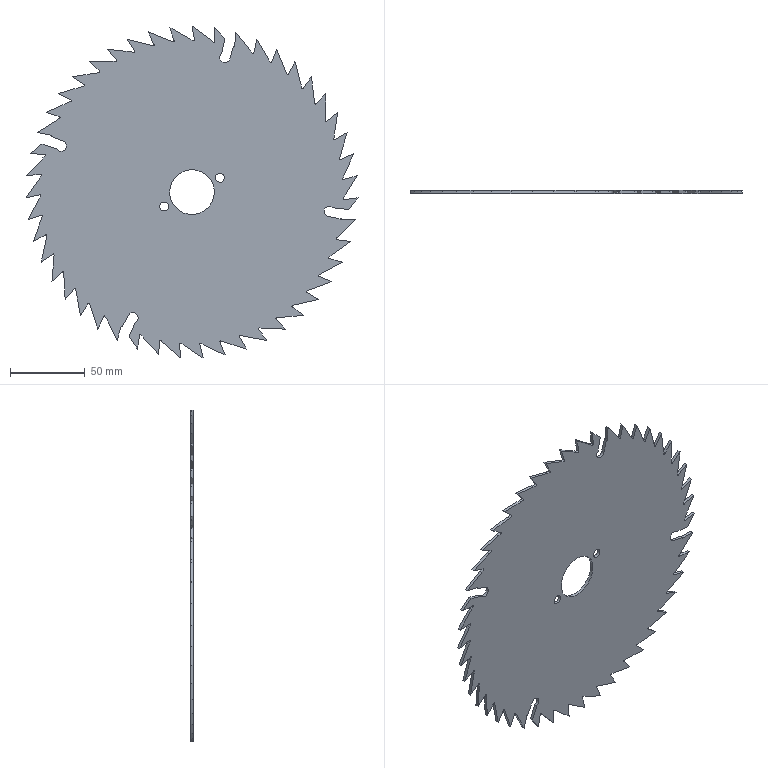Component | SolidWorks | Blade-1 | 1 solid | 163 faces | box 222.59 x 2 x 222.47 mm | volume 68140 mm3 | plane 104 | spline 47 | cylinder 12 | commonest cylinder face diameters 7 x6 6 x4 30 x2